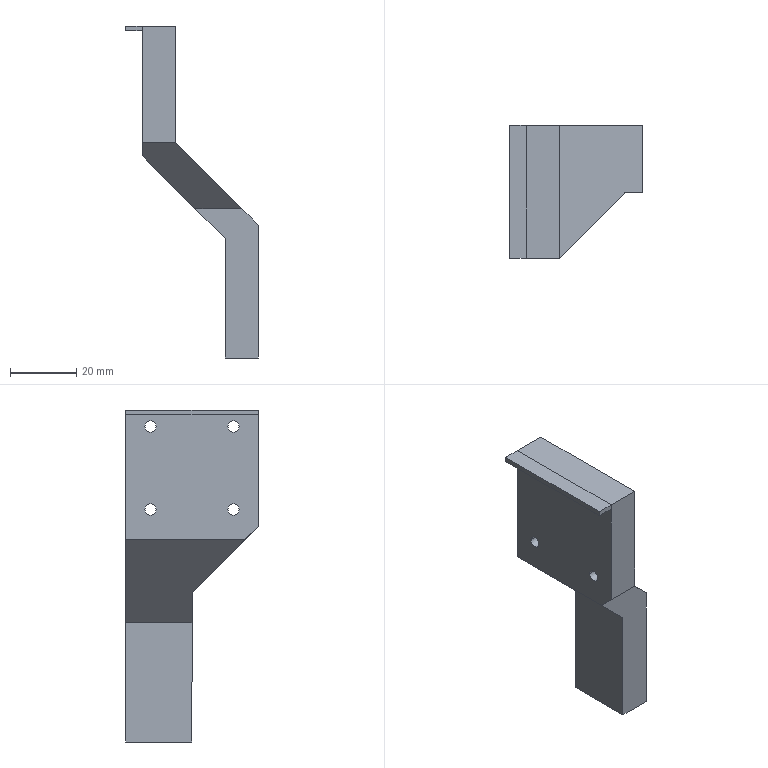Component | SolidWorks | Slider-1 | 2 solids | 26 faces | box 40 x 40 x 100 mm | volume 31677 mm3 | plane 18 | cylinder 8 | commonest cylinder face diameters 3.4 x8
STEP:
#1=COLOUR_RGB('',0.7922,0.8196,0.9333);
#2=FILL_AREA_STYLE_COLOUR('',#1);
#3=FILL_AREA_STYLE('',(#2));
#4=SURFACE_STYLE_FILL_AREA(#3);
#5=SURFACE_SIDE_STYLE('',(#4));
#6=SURFACE_STYLE_USAGE(.BOTH.,#5);
#7=PRESENTATION_STYLE_ASSIGNMENT((#6));
#8=CARTESIAN_POINT('',(-23.049,0.5207,17.664));
#9=VERTEX_POINT('',#8);
#10=CARTESIAN_POINT('',(-23.049,0.6546,17.664));
#11=VERTEX_POINT('',#10);
#12=CARTESIAN_POINT('',(-23.049,0.5877,17.664));
#13=DIRECTION('',(-1.,-0.,-0.));
#14=DIRECTION('',(0.,1.,0.));
#15=AXIS2_PLACEMENT_3D('',#12,#13,#14);
#16=CIRCLE('',#15,0.06693);
#17=EDGE_CURVE('',#9,#11,#16,.T.);
#18=ORIENTED_EDGE('',*,*,#17,.T.);
#19=CARTESIAN_POINT('',(-22.655,0.6546,17.664));
#20=VERTEX_POINT('',#19);
#21=CARTESIAN_POINT('',(-21.671,0.6546,17.664));
#22=DIRECTION('',(1.,0.,0.));
#23=VECTOR('',#22,39.37);
#24=LINE('',#21,#23);
#25=EDGE_CURVE('',#11,#20,#24,.T.);
#26=ORIENTED_EDGE('',*,*,#25,.T.);
#27=CARTESIAN_POINT('',(-22.655,0.5207,17.664));
#28=VERTEX_POINT('',#27);
#29=CARTESIAN_POINT('',(-22.655,0.5877,17.664));
#30=DIRECTION('',(-1.,-0.,-0.));
#31=DIRECTION('',(0.,-1.,0.));
#32=AXIS2_PLACEMENT_3D('',#29,#30,#31);
#33=CIRCLE('',#32,0.06693);
#34=EDGE_CURVE('',#28,#20,#33,.T.);
#35=ORIENTED_EDGE('',*,*,#34,.F.);
#36=CARTESIAN_POINT('',(-21.671,0.5207,17.664));
#37=DIRECTION('',(1.,0.,0.));
#38=VECTOR('',#37,39.37);
#39=LINE('',#36,#38);
#40=EDGE_CURVE('',#9,#28,#39,.T.);
#41=ORIENTED_EDGE('',*,*,#40,.F.);
#42=EDGE_LOOP('',(#18,#26,#35,#41));
#43=FACE_OUTER_BOUND('',#42,.T.);
#44=CARTESIAN_POINT('',(-21.671,0.5877,17.664));
#45=DIRECTION('',(1.,0.,0.));
#46=DIRECTION('',(0.,-1.,0.));
#47=AXIS2_PLACEMENT_3D('',#44,#45,#46);
#48=CYLINDRICAL_SURFACE('',#47,0.06693);
#49=ADVANCED_FACE('',(#43),#48,.F.);
#50=CARTESIAN_POINT('',(-23.049,-0.4635,17.664));
#51=VERTEX_POINT('',#50);
#52=CARTESIAN_POINT('',(-23.049,-0.3297,17.664));
#53=VERTEX_POINT('',#52);
#54=CARTESIAN_POINT('',(-23.049,-0.3966,17.664));
#55=DIRECTION('',(-1.,-0.,-0.));
#56=DIRECTION('',(0.,1.,0.));
#57=AXIS2_PLACEMENT_3D('',#54,#55,#56);
#58=CIRCLE('',#57,0.06693);
#59=EDGE_CURVE('',#51,#53,#58,.T.);
#60=ORIENTED_EDGE('',*,*,#59,.T.);
#61=CARTESIAN_POINT('',(-22.655,-0.3297,17.664));
#62=VERTEX_POINT('',#61);
#63=CARTESIAN_POINT('',(-21.671,-0.3297,17.664));
#64=DIRECTION('',(1.,0.,0.));
#65=VECTOR('',#64,39.37);
#66=LINE('',#63,#65);
#67=EDGE_CURVE('',#53,#62,#66,.T.);
#68=ORIENTED_EDGE('',*,*,#67,.T.);
#69=CARTESIAN_POINT('',(-22.655,-0.4635,17.664));
#70=VERTEX_POINT('',#69);
#71=CARTESIAN_POINT('',(-22.655,-0.3966,17.664));
#72=DIRECTION('',(-1.,-0.,-0.));
#73=DIRECTION('',(0.,-1.,0.));
#74=AXIS2_PLACEMENT_3D('',#71,#72,#73);
#75=CIRCLE('',#74,0.06693);
#76=EDGE_CURVE('',#70,#62,#75,.T.);
#77=ORIENTED_EDGE('',*,*,#76,.F.);
#78=CARTESIAN_POINT('',(-21.671,-0.4635,17.664));
#79=DIRECTION('',(1.,0.,0.));
#80=VECTOR('',#79,39.37);
#81=LINE('',#78,#80);
#82=EDGE_CURVE('',#51,#70,#81,.T.);
#83=ORIENTED_EDGE('',*,*,#82,.F.);
#84=EDGE_LOOP('',(#60,#68,#77,#83));
#85=FACE_OUTER_BOUND('',#84,.T.);
#86=CARTESIAN_POINT('',(-21.671,-0.3966,17.664));
#87=DIRECTION('',(1.,0.,0.));
#88=DIRECTION('',(0.,-1.,0.));
#89=AXIS2_PLACEMENT_3D('',#86,#87,#88);
#90=CYLINDRICAL_SURFACE('',#89,0.06693);
#91=ADVANCED_FACE('',(#85),#90,.F.);
#92=CARTESIAN_POINT('',(-23.049,0.5207,16.68));
#93=VERTEX_POINT('',#92);
#94=CARTESIAN_POINT('',(-23.049,0.6546,16.68));
#95=VERTEX_POINT('',#94);
#96=CARTESIAN_POINT('',(-23.049,0.5877,16.68));
#97=DIRECTION('',(-1.,-0.,-0.));
#98=DIRECTION('',(0.,1.,0.));
#99=AXIS2_PLACEMENT_3D('',#96,#97,#98);
#100=CIRCLE('',#99,0.06693);
#101=EDGE_CURVE('',#93,#95,#100,.T.);
#102=ORIENTED_EDGE('',*,*,#101,.T.);
#103=CARTESIAN_POINT('',(-22.655,0.6546,16.68));
#104=VERTEX_POINT('',#103);
#105=CARTESIAN_POINT('',(-21.671,0.6546,16.68));
#106=DIRECTION('',(1.,0.,0.));
#107=VECTOR('',#106,39.37);
#108=LINE('',#105,#107);
#109=EDGE_CURVE('',#95,#104,#108,.T.);
#110=ORIENTED_EDGE('',*,*,#109,.T.);
#111=CARTESIAN_POINT('',(-22.655,0.5207,16.68));
#112=VERTEX_POINT('',#111);
#113=CARTESIAN_POINT('',(-22.655,0.5877,16.68));
#114=DIRECTION('',(-1.,-0.,-0.));
#115=DIRECTION('',(0.,-1.,0.));
#116=AXIS2_PLACEMENT_3D('',#113,#114,#115);
#117=CIRCLE('',#116,0.06693);
#118=EDGE_CURVE('',#112,#104,#117,.T.);
#119=ORIENTED_EDGE('',*,*,#118,.F.);
#120=CARTESIAN_POINT('',(-21.671,0.5207,16.68));
#121=DIRECTION('',(1.,0.,0.));
#122=VECTOR('',#121,39.37);
#123=LINE('',#120,#122);
#124=EDGE_CURVE('',#93,#112,#123,.T.);
#125=ORIENTED_EDGE('',*,*,#124,.F.);
#126=EDGE_LOOP('',(#102,#110,#119,#125));
#127=FACE_OUTER_BOUND('',#126,.T.);
#128=CARTESIAN_POINT('',(-21.671,0.5877,16.68));
#129=DIRECTION('',(1.,0.,0.));
#130=DIRECTION('',(0.,-1.,0.));
#131=AXIS2_PLACEMENT_3D('',#128,#129,#130);
#132=CYLINDRICAL_SURFACE('',#131,0.06693);
#133=ADVANCED_FACE('',(#127),#132,.F.);
#134=CARTESIAN_POINT('',(-23.049,-0.4635,16.68));
#135=VERTEX_POINT('',#134);
#136=CARTESIAN_POINT('',(-23.049,-0.3297,16.68));
#137=VERTEX_POINT('',#136);
#138=CARTESIAN_POINT('',(-23.049,-0.3966,16.68));
#139=DIRECTION('',(-1.,-0.,-0.));
#140=DIRECTION('',(0.,1.,0.));
#141=AXIS2_PLACEMENT_3D('',#138,#139,#140);
#142=CIRCLE('',#141,0.06693);
#143=EDGE_CURVE('',#135,#137,#142,.T.);
#144=ORIENTED_EDGE('',*,*,#143,.T.);
#145=CARTESIAN_POINT('',(-22.655,-0.3297,16.68));
#146=VERTEX_POINT('',#145);
#147=CARTESIAN_POINT('',(-21.671,-0.3297,16.68));
#148=DIRECTION('',(1.,0.,0.));
#149=VECTOR('',#148,39.37);
#150=LINE('',#147,#149);
#151=EDGE_CURVE('',#137,#146,#150,.T.);
#152=ORIENTED_EDGE('',*,*,#151,.T.);
#153=CARTESIAN_POINT('',(-22.655,-0.4635,16.68));
#154=VERTEX_POINT('',#153);
#155=CARTESIAN_POINT('',(-22.655,-0.3966,16.68));
#156=DIRECTION('',(-1.,-0.,-0.));
#157=DIRECTION('',(0.,-1.,0.));
#158=AXIS2_PLACEMENT_3D('',#155,#156,#157);
#159=CIRCLE('',#158,0.06693);
#160=EDGE_CURVE('',#154,#146,#159,.T.);
#161=ORIENTED_EDGE('',*,*,#160,.F.);
#162=CARTESIAN_POINT('',(-21.671,-0.4635,16.68));
#163=DIRECTION('',(1.,0.,0.));
#164=VECTOR('',#163,39.37);
#165=LINE('',#162,#164);
#166=EDGE_CURVE('',#135,#154,#165,.T.);
#167=ORIENTED_EDGE('',*,*,#166,.F.);
#168=EDGE_LOOP('',(#144,#152,#161,#167));
#169=FACE_OUTER_BOUND('',#168,.T.);
#170=CARTESIAN_POINT('',(-21.671,-0.3966,16.68));
#171=DIRECTION('',(1.,0.,0.));
#172=DIRECTION('',(0.,-1.,0.));
#173=AXIS2_PLACEMENT_3D('',#170,#171,#172);
#174=CYLINDRICAL_SURFACE('',#173,0.06693);
#175=ADVANCED_FACE('',(#169),#174,.F.);
#176=CARTESIAN_POINT('',(-22.655,0.8829,17.861));
#177=VERTEX_POINT('',#176);
#178=CARTESIAN_POINT('',(-22.655,0.8829,16.483));
#179=VERTEX_POINT('',#178);
#180=CARTESIAN_POINT('',(-22.655,0.8829,17.861));
#181=DIRECTION('',(0.,0.,-1.));
#182=VECTOR('',#181,39.37);
#183=LINE('',#180,#182);
#184=EDGE_CURVE('',#177,#179,#183,.T.);
#185=ORIENTED_EDGE('',*,*,#184,.T.);
#186=CARTESIAN_POINT('',(-21.671,0.8829,15.499));
#187=VERTEX_POINT('',#186);
#188=CARTESIAN_POINT('',(-22.655,0.8829,16.483));
#189=DIRECTION('',(0.7071,0.,-0.7071));
#190=VECTOR('',#189,39.37);
#191=LINE('',#188,#190);
#192=EDGE_CURVE('',#179,#187,#191,.T.);
#193=ORIENTED_EDGE('',*,*,#192,.T.);
#194=CARTESIAN_POINT('',(-21.671,0.8829,13.924));
#195=VERTEX_POINT('',#194);
#196=CARTESIAN_POINT('',(-21.671,0.8829,17.861));
#197=DIRECTION('',(-0.,-0.,1.));
#198=VECTOR('',#197,39.37);
#199=LINE('',#196,#198);
#200=EDGE_CURVE('',#195,#187,#199,.T.);
#201=ORIENTED_EDGE('',*,*,#200,.F.);
#202=CARTESIAN_POINT('',(-22.065,0.8829,13.924));
#203=VERTEX_POINT('',#202);
#204=CARTESIAN_POINT('',(-21.671,0.8829,13.924));
#205=DIRECTION('',(-1.,-0.,-0.));
#206=VECTOR('',#205,39.37);
#207=LINE('',#204,#206);
#208=EDGE_CURVE('',#195,#203,#207,.T.);
#209=ORIENTED_EDGE('',*,*,#208,.T.);
#210=CARTESIAN_POINT('',(-22.065,0.8829,15.336));
#211=VERTEX_POINT('',#210);
#212=CARTESIAN_POINT('',(-22.065,0.8829,13.924));
#213=DIRECTION('',(-0.,-0.,1.));
#214=VECTOR('',#213,39.37);
#215=LINE('',#212,#214);
#216=EDGE_CURVE('',#203,#211,#215,.T.);
#217=ORIENTED_EDGE('',*,*,#216,.T.);
#218=CARTESIAN_POINT('',(-23.049,0.8829,16.32));
#219=VERTEX_POINT('',#218);
#220=CARTESIAN_POINT('',(-22.065,0.8829,15.336));
#221=DIRECTION('',(-0.7071,-0.,0.7071));
#222=VECTOR('',#221,39.37);
#223=LINE('',#220,#222);
#224=EDGE_CURVE('',#211,#219,#223,.T.);
#225=ORIENTED_EDGE('',*,*,#224,.T.);
#226=CARTESIAN_POINT('',(-23.049,0.8829,17.861));
#227=VERTEX_POINT('',#226);
#228=CARTESIAN_POINT('',(-23.049,0.8829,17.861));
#229=DIRECTION('',(-0.,-0.,1.));
#230=VECTOR('',#229,39.37);
#231=LINE('',#228,#230);
#232=EDGE_CURVE('',#219,#227,#231,.T.);
#233=ORIENTED_EDGE('',*,*,#232,.T.);
#234=CARTESIAN_POINT('',(-21.671,0.8829,17.861));
#235=DIRECTION('',(-1.,-0.,-0.));
#236=VECTOR('',#235,39.37);
#237=LINE('',#234,#236);
#238=EDGE_CURVE('',#177,#227,#237,.T.);
#239=ORIENTED_EDGE('',*,*,#238,.F.);
#240=EDGE_LOOP('',(#185,#193,#201,#209,#217,#225,#233,#239));
#241=FACE_OUTER_BOUND('',#240,.T.);
#242=CARTESIAN_POINT('',(-21.671,0.8829,17.861));
#243=DIRECTION('',(0.,-1.,-0.));
#244=DIRECTION('',(-1.,-0.,-0.));
#245=AXIS2_PLACEMENT_3D('',#242,#243,#244);
#246=PLANE('',#245);
#247=ADVANCED_FACE('',(#241),#246,.F.);
#248=CARTESIAN_POINT('',(-22.655,-0.6919,17.861));
#249=VERTEX_POINT('',#248);
#250=CARTESIAN_POINT('',(-22.655,-1.282,17.861));
#251=DIRECTION('',(-0.,1.,0.));
#252=VECTOR('',#251,39.37);
#253=LINE('',#250,#252);
#254=EDGE_CURVE('',#249,#177,#253,.T.);
#255=ORIENTED_EDGE('',*,*,#254,.T.);
#256=ORIENTED_EDGE('',*,*,#238,.T.);
#257=CARTESIAN_POINT('',(-23.049,-0.6919,17.861));
#258=VERTEX_POINT('',#257);
#259=CARTESIAN_POINT('',(-23.049,0.8829,17.861));
#260=DIRECTION('',(0.,-1.,-0.));
#261=VECTOR('',#260,39.37);
#262=LINE('',#259,#261);
#263=EDGE_CURVE('',#227,#258,#262,.T.);
#264=ORIENTED_EDGE('',*,*,#263,.T.);
#265=CARTESIAN_POINT('',(-21.671,-0.6919,17.861));
#266=DIRECTION('',(-1.,-0.,-0.));
#267=VECTOR('',#266,39.37);
#268=LINE('',#265,#267);
#269=EDGE_CURVE('',#249,#258,#268,.T.);
#270=ORIENTED_EDGE('',*,*,#269,.F.);
#271=EDGE_LOOP('',(#255,#256,#264,#270));
#272=FACE_OUTER_BOUND('',#271,.T.);
#273=CARTESIAN_POINT('',(-21.671,0.8829,17.861));
#274=DIRECTION('',(0.,0.,-1.));
#275=DIRECTION('',(1.,0.,0.));
#276=AXIS2_PLACEMENT_3D('',#273,#274,#275);
#277=PLANE('',#276);
#278=ADVANCED_FACE('',(#272),#277,.F.);
#279=CARTESIAN_POINT('',(-22.655,-0.6919,16.483));
#280=VERTEX_POINT('',#279);
#281=CARTESIAN_POINT('',(-22.655,-0.6919,17.861));
#282=DIRECTION('',(0.,0.,-1.));
#283=VECTOR('',#282,39.37);
#284=LINE('',#281,#283);
#285=EDGE_CURVE('',#249,#280,#284,.T.);
#286=ORIENTED_EDGE('',*,*,#285,.F.);
#287=ORIENTED_EDGE('',*,*,#269,.T.);
#288=CARTESIAN_POINT('',(-23.049,-0.6919,16.483));
#289=VERTEX_POINT('',#288);
#290=CARTESIAN_POINT('',(-23.049,-0.6919,17.861));
#291=DIRECTION('',(0.,0.,-1.));
#292=VECTOR('',#291,39.37);
#293=LINE('',#290,#292);
#294=EDGE_CURVE('',#258,#289,#293,.T.);
#295=ORIENTED_EDGE('',*,*,#294,.T.);
#296=CARTESIAN_POINT('',(-21.671,-0.6919,16.483));
#297=DIRECTION('',(-1.,-0.,-0.));
#298=VECTOR('',#297,39.37);
#299=LINE('',#296,#298);
#300=EDGE_CURVE('',#280,#289,#299,.T.);
#301=ORIENTED_EDGE('',*,*,#300,.F.);
#302=EDGE_LOOP('',(#286,#287,#295,#301));
#303=FACE_OUTER_BOUND('',#302,.T.);
#304=CARTESIAN_POINT('',(-21.671,-0.6919,17.861));
#305=DIRECTION('',(-0.,1.,0.));
#306=DIRECTION('',(-0.,-0.,1.));
#307=AXIS2_PLACEMENT_3D('',#304,#305,#306);
#308=PLANE('',#307);
#309=ADVANCED_FACE('',(#303),#308,.F.);
#310=CARTESIAN_POINT('',(-21.868,0.09553,15.696));
#311=VERTEX_POINT('',#310);
#312=CARTESIAN_POINT('',(-21.671,0.09553,15.499));
#313=VERTEX_POINT('',#312);
#314=CARTESIAN_POINT('',(-22.163,0.09553,15.991));
#315=DIRECTION('',(0.7071,0.,-0.7071));
#316=VECTOR('',#315,39.37);
#317=LINE('',#314,#316);
#318=EDGE_CURVE('',#311,#313,#317,.T.);
#319=ORIENTED_EDGE('',*,*,#318,.F.);
#320=CARTESIAN_POINT('',(-22.425,0.09553,15.696));
#321=VERTEX_POINT('',#320);
#322=CARTESIAN_POINT('',(-23.049,0.09553,15.696));
#323=DIRECTION('',(-1.,-0.,-0.));
#324=VECTOR('',#323,39.37);
#325=LINE('',#322,#324);
#326=EDGE_CURVE('',#311,#321,#325,.T.);
#327=ORIENTED_EDGE('',*,*,#326,.T.);
#328=CARTESIAN_POINT('',(-22.065,0.09553,15.336));
#329=VERTEX_POINT('',#328);
#330=CARTESIAN_POINT('',(-22.442,0.09553,15.712));
#331=DIRECTION('',(-0.7071,-0.,0.7071));
#332=VECTOR('',#331,39.37);
#333=LINE('',#330,#332);
#334=EDGE_CURVE('',#329,#321,#333,.T.);
#335=ORIENTED_EDGE('',*,*,#334,.F.);
#336=CARTESIAN_POINT('',(-22.065,0.09553,13.924));
#337=VERTEX_POINT('',#336);
#338=CARTESIAN_POINT('',(-22.065,0.09553,16.483));
#339=DIRECTION('',(-0.,-0.,1.));
#340=VECTOR('',#339,39.37);
#341=LINE('',#338,#340);
#342=EDGE_CURVE('',#337,#329,#341,.T.);
#343=ORIENTED_EDGE('',*,*,#342,.F.);
#344=CARTESIAN_POINT('',(-21.671,0.09553,13.924));
#345=VERTEX_POINT('',#344);
#346=CARTESIAN_POINT('',(-21.671,0.09553,13.924));
#347=DIRECTION('',(-1.,-0.,-0.));
#348=VECTOR('',#347,39.37);
#349=LINE('',#346,#348);
#350=EDGE_CURVE('',#345,#337,#349,.T.);
#351=ORIENTED_EDGE('',*,*,#350,.F.);
#352=CARTESIAN_POINT('',(-21.671,0.09553,16.483));
#353=DIRECTION('',(0.,0.,-1.));
#354=VECTOR('',#353,39.37);
#355=LINE('',#352,#354);
#356=EDGE_CURVE('',#313,#345,#355,.T.);
#357=ORIENTED_EDGE('',*,*,#356,.F.);
#358=EDGE_LOOP('',(#319,#327,#335,#343,#351,#357));
#359=FACE_OUTER_BOUND('',#358,.T.);
#360=CARTESIAN_POINT('',(-21.671,0.09553,16.483));
#361=DIRECTION('',(-0.,1.,0.));
#362=DIRECTION('',(1.,0.,0.));
#363=AXIS2_PLACEMENT_3D('',#360,#361,#362);
#364=PLANE('',#363);
#365=ADVANCED_FACE('',(#359),#364,.F.);
#366=CARTESIAN_POINT('',(-22.065,-1.282,13.924));
#367=DIRECTION('',(-0.,1.,0.));
#368=VECTOR('',#367,39.37);
#369=LINE('',#366,#368);
#370=EDGE_CURVE('',#337,#203,#369,.T.);
#371=ORIENTED_EDGE('',*,*,#370,.T.);
#372=ORIENTED_EDGE('',*,*,#208,.F.);
#373=CARTESIAN_POINT('',(-21.671,0.8829,13.924));
#374=DIRECTION('',(-0.,1.,0.));
#375=VECTOR('',#374,39.37);
#376=LINE('',#373,#375);
#377=EDGE_CURVE('',#345,#195,#376,.T.);
#378=ORIENTED_EDGE('',*,*,#377,.F.);
#379=ORIENTED_EDGE('',*,*,#350,.T.);
#380=EDGE_LOOP('',(#371,#372,#378,#379));
#381=FACE_OUTER_BOUND('',#380,.T.);
#382=CARTESIAN_POINT('',(-21.671,0.8829,13.924));
#383=DIRECTION('',(-0.,-0.,1.));
#384=DIRECTION('',(-1.,-0.,-0.));
#385=AXIS2_PLACEMENT_3D('',#382,#383,#384);
#386=PLANE('',#385);
#387=ADVANCED_FACE('',(#381),#386,.F.);
#388=CARTESIAN_POINT('',(-21.671,-1.282,15.499));
#389=DIRECTION('',(-0.,1.,0.));
#390=VECTOR('',#389,39.37);
#391=LINE('',#388,#390);
#392=EDGE_CURVE('',#313,#187,#391,.T.);
#393=ORIENTED_EDGE('',*,*,#392,.F.);
#394=ORIENTED_EDGE('',*,*,#356,.T.);
#395=ORIENTED_EDGE('',*,*,#377,.T.);
#396=ORIENTED_EDGE('',*,*,#200,.T.);
#397=EDGE_LOOP('',(#393,#394,#395,#396));
#398=FACE_OUTER_BOUND('',#397,.T.);
#399=CARTESIAN_POINT('',(-21.671,0.1353,17.169));
#400=DIRECTION('',(-1.,-0.,-0.));
#401=DIRECTION('',(-0.,1.,0.));
#402=AXIS2_PLACEMENT_3D('',#399,#400,#401);
#403=PLANE('',#402);
#404=ADVANCED_FACE('',(#398),#403,.F.);
#405=ORIENTED_EDGE('',*,*,#17,.F.);
#406=CARTESIAN_POINT('',(-23.049,0.5877,17.664));
#407=DIRECTION('',(-1.,-0.,-0.));
#408=DIRECTION('',(0.,1.,0.));
#409=AXIS2_PLACEMENT_3D('',#406,#407,#408);
#410=CIRCLE('',#409,0.06693);
#411=EDGE_CURVE('',#11,#9,#410,.T.);
#412=ORIENTED_EDGE('',*,*,#411,.F.);
#413=EDGE_LOOP('',(#405,#412));
#414=FACE_BOUND('',#413,.T.);
#415=ORIENTED_EDGE('',*,*,#59,.F.);
#416=CARTESIAN_POINT('',(-23.049,-0.3966,17.664));
#417=DIRECTION('',(-1.,-0.,-0.));
#418=DIRECTION('',(0.,1.,0.));
#419=AXIS2_PLACEMENT_3D('',#416,#417,#418);
#420=CIRCLE('',#419,0.06693);
#421=EDGE_CURVE('',#53,#51,#420,.T.);
#422=ORIENTED_EDGE('',*,*,#421,.F.);
#423=EDGE_LOOP('',(#415,#422));
#424=FACE_BOUND('',#423,.T.);
#425=ORIENTED_EDGE('',*,*,#101,.F.);
#426=CARTESIAN_POINT('',(-23.049,0.5877,16.68));
#427=DIRECTION('',(-1.,-0.,-0.));
#428=DIRECTION('',(0.,1.,0.));
#429=AXIS2_PLACEMENT_3D('',#426,#427,#428);
#430=CIRCLE('',#429,0.06693);
#431=EDGE_CURVE('',#95,#93,#430,.T.);
#432=ORIENTED_EDGE('',*,*,#431,.F.);
#433=EDGE_LOOP('',(#425,#432));
#434=FACE_BOUND('',#433,.T.);
#435=ORIENTED_EDGE('',*,*,#143,.F.);
#436=CARTESIAN_POINT('',(-23.049,-0.3966,16.68));
#437=DIRECTION('',(-1.,-0.,-0.));
#438=DIRECTION('',(0.,1.,0.));
#439=AXIS2_PLACEMENT_3D('',#436,#437,#438);
#440=CIRCLE('',#439,0.06693);
#441=EDGE_CURVE('',#137,#135,#440,.T.);
#442=ORIENTED_EDGE('',*,*,#441,.F.);
#443=EDGE_LOOP('',(#435,#442));
#444=FACE_BOUND('',#443,.T.);
#445=ORIENTED_EDGE('',*,*,#232,.F.);
#446=CARTESIAN_POINT('',(-23.049,-0.5288,16.32));
#447=VERTEX_POINT('',#446);
#448=CARTESIAN_POINT('',(-23.049,-1.282,16.32));
#449=DIRECTION('',(-0.,1.,0.));
#450=VECTOR('',#449,39.37);
#451=LINE('',#448,#450);
#452=EDGE_CURVE('',#447,#219,#451,.T.);
#453=ORIENTED_EDGE('',*,*,#452,.F.);
#454=CARTESIAN_POINT('',(-23.049,0.09553,15.696));
#455=DIRECTION('',(-0.,-0.7071,0.7071));
#456=VECTOR('',#455,39.37);
#457=LINE('',#454,#456);
#458=EDGE_CURVE('',#447,#289,#457,.T.);
#459=ORIENTED_EDGE('',*,*,#458,.T.);
#460=ORIENTED_EDGE('',*,*,#294,.F.);
#461=ORIENTED_EDGE('',*,*,#263,.F.);
#462=EDGE_LOOP('',(#445,#453,#459,#460,#461));
#463=FACE_OUTER_BOUND('',#462,.T.);
#464=CARTESIAN_POINT('',(-23.049,0.1353,17.169));
#465=DIRECTION('',(-1.,-0.,-0.));
#466=DIRECTION('',(-0.,1.,0.));
#467=AXIS2_PLACEMENT_3D('',#464,#465,#466);
#468=PLANE('',#467);
#469=ADVANCED_FACE('',(#414,#424,#434,#444,#463),#468,.T.);
#470=CARTESIAN_POINT('',(-21.802,0.1611,15.63));
#471=DIRECTION('',(0.5774,0.5774,-0.5774));
#472=VECTOR('',#471,39.37);
#473=LINE('',#470,#472);
#474=EDGE_CURVE('',#280,#311,#473,.T.);
#475=ORIENTED_EDGE('',*,*,#474,.F.);
#476=ORIENTED_EDGE('',*,*,#300,.T.);
#477=ORIENTED_EDGE('',*,*,#458,.F.);
#478=CARTESIAN_POINT('',(-22.174,0.3467,15.444));
#479=DIRECTION('',(-0.5774,-0.5774,0.5774));
#480=VECTOR('',#479,39.37);
#481=LINE('',#478,#480);
#482=EDGE_CURVE('',#321,#447,#481,.T.);
#483=ORIENTED_EDGE('',*,*,#482,.F.);
#484=ORIENTED_EDGE('',*,*,#326,.F.);
#485=EDGE_LOOP('',(#475,#476,#477,#483,#484));
#486=FACE_OUTER_BOUND('',#485,.T.);
#487=CARTESIAN_POINT('',(-21.671,0.09553,15.696));
#488=DIRECTION('',(0.,-0.7071,-0.7071));
#489=DIRECTION('',(1.,0.,0.));
#490=AXIS2_PLACEMENT_3D('',#487,#488,#489);
#491=PLANE('',#490);
#492=ADVANCED_FACE('',(#486),#491,.T.);
#493=ORIENTED_EDGE('',*,*,#151,.F.);
#494=ORIENTED_EDGE('',*,*,#441,.T.);
#495=ORIENTED_EDGE('',*,*,#166,.T.);
#496=CARTESIAN_POINT('',(-22.655,-0.3966,16.68));
#497=DIRECTION('',(-1.,-0.,-0.));
#498=DIRECTION('',(0.,-1.,0.));
#499=AXIS2_PLACEMENT_3D('',#496,#497,#498);
#500=CIRCLE('',#499,0.06693);
#501=EDGE_CURVE('',#146,#154,#500,.T.);
#502=ORIENTED_EDGE('',*,*,#501,.F.);
#503=EDGE_LOOP('',(#493,#494,#495,#502));
#504=FACE_OUTER_BOUND('',#503,.T.);
#505=CARTESIAN_POINT('',(-21.671,-0.3966,16.68));
#506=DIRECTION('',(1.,0.,0.));
#507=DIRECTION('',(0.,-1.,0.));
#508=AXIS2_PLACEMENT_3D('',#505,#506,#507);
#509=CYLINDRICAL_SURFACE('',#508,0.06693);
#510=ADVANCED_FACE('',(#504),#509,.F.);
#511=ORIENTED_EDGE('',*,*,#109,.F.);
#512=ORIENTED_EDGE('',*,*,#431,.T.);
#513=ORIENTED_EDGE('',*,*,#124,.T.);
#514=CARTESIAN_POINT('',(-22.655,0.5877,16.68));
#515=DIRECTION('',(-1.,-0.,-0.));
#516=DIRECTION('',(0.,-1.,0.));
#517=AXIS2_PLACEMENT_3D('',#514,#515,#516);
#518=CIRCLE('',#517,0.06693);
#519=EDGE_CURVE('',#104,#112,#518,.T.);
#520=ORIENTED_EDGE('',*,*,#519,.F.);
#521=EDGE_LOOP('',(#511,#512,#513,#520));
#522=FACE_OUTER_BOUND('',#521,.T.);
#523=CARTESIAN_POINT('',(-21.671,0.5877,16.68));
#524=DIRECTION('',(1.,0.,0.));
#525=DIRECTION('',(0.,-1.,0.));
#526=AXIS2_PLACEMENT_3D('',#523,#524,#525);
#527=CYLINDRICAL_SURFACE('',#526,0.06693);
#528=ADVANCED_FACE('',(#522),#527,.F.);
#529=ORIENTED_EDGE('',*,*,#67,.F.);
#530=ORIENTED_EDGE('',*,*,#421,.T.);
#531=ORIENTED_EDGE('',*,*,#82,.T.);
#532=CARTESIAN_POINT('',(-22.655,-0.3966,17.664));
#533=DIRECTION('',(-1.,-0.,-0.));
#534=DIRECTION('',(0.,-1.,0.));
#535=AXIS2_PLACEMENT_3D('',#532,#533,#534);
#536=CIRCLE('',#535,0.06693);
#537=EDGE_CURVE('',#62,#70,#536,.T.);
#538=ORIENTED_EDGE('',*,*,#537,.F.);
#539=EDGE_LOOP('',(#529,#530,#531,#538));
#540=FACE_OUTER_BOUND('',#539,.T.);
#541=CARTESIAN_POINT('',(-21.671,-0.3966,17.664));
#542=DIRECTION('',(1.,0.,0.));
#543=DIRECTION('',(0.,-1.,0.));
#544=AXIS2_PLACEMENT_3D('',#541,#542,#543);
#545=CYLINDRICAL_SURFACE('',#544,0.06693);
#546=ADVANCED_FACE('',(#540),#545,.F.);
#547=ORIENTED_EDGE('',*,*,#25,.F.);
#548=ORIENTED_EDGE('',*,*,#411,.T.);
#549=ORIENTED_EDGE('',*,*,#40,.T.);
#550=CARTESIAN_POINT('',(-22.655,0.5877,17.664));
#551=DIRECTION('',(-1.,-0.,-0.));
#552=DIRECTION('',(0.,-1.,0.));
#553=AXIS2_PLACEMENT_3D('',#550,#551,#552);
#554=CIRCLE('',#553,0.06693);
#555=EDGE_CURVE('',#20,#28,#554,.T.);
#556=ORIENTED_EDGE('',*,*,#555,.F.);
#557=EDGE_LOOP('',(#547,#548,#549,#556));
#558=FACE_OUTER_BOUND('',#557,.T.);
#559=CARTESIAN_POINT('',(-21.671,0.5877,17.664));
#560=DIRECTION('',(1.,0.,0.));
#561=DIRECTION('',(0.,-1.,0.));
#562=AXIS2_PLACEMENT_3D('',#559,#560,#561);
#563=CYLINDRICAL_SURFACE('',#562,0.06693);
#564=ADVANCED_FACE('',(#558),#563,.F.);
#565=ORIENTED_EDGE('',*,*,#318,.T.);
#566=ORIENTED_EDGE('',*,*,#392,.T.);
#567=ORIENTED_EDGE('',*,*,#192,.F.);
#568=CARTESIAN_POINT('',(-22.655,-1.282,16.483));
#569=DIRECTION('',(-0.,1.,0.));
#570=VECTOR('',#569,39.37);
#571=LINE('',#568,#570);
#572=EDGE_CURVE('',#280,#179,#571,.T.);
#573=ORIENTED_EDGE('',*,*,#572,.F.);
#574=ORIENTED_EDGE('',*,*,#474,.T.);
#575=EDGE_LOOP('',(#565,#566,#567,#573,#574));
#576=FACE_OUTER_BOUND('',#575,.T.);
#577=CARTESIAN_POINT('',(-22.655,-1.282,16.483));
#578=DIRECTION('',(0.7071,-0.,0.7071));
#579=DIRECTION('',(-0.7071,-0.,0.7071));
#580=AXIS2_PLACEMENT_3D('',#577,#578,#579);
#581=PLANE('',#580);
#582=ADVANCED_FACE('',(#576),#581,.T.);
#583=ORIENTED_EDGE('',*,*,#160,.T.);
#584=ORIENTED_EDGE('',*,*,#501,.T.);
#585=EDGE_LOOP('',(#583,#584));
#586=FACE_BOUND('',#585,.T.);
#587=ORIENTED_EDGE('',*,*,#118,.T.);
#588=ORIENTED_EDGE('',*,*,#519,.T.);
#589=EDGE_LOOP('',(#587,#588));
#590=FACE_BOUND('',#589,.T.);
#591=ORIENTED_EDGE('',*,*,#76,.T.);
#592=ORIENTED_EDGE('',*,*,#537,.T.);
#593=EDGE_LOOP('',(#591,#592));
#594=FACE_BOUND('',#593,.T.);
#595=ORIENTED_EDGE('',*,*,#34,.T.);
#596=ORIENTED_EDGE('',*,*,#555,.T.);
#597=EDGE_LOOP('',(#595,#596));
#598=FACE_BOUND('',#597,.T.);
#599=ORIENTED_EDGE('',*,*,#285,.T.);
#600=ORIENTED_EDGE('',*,*,#572,.T.);
#601=ORIENTED_EDGE('',*,*,#184,.F.);
#602=ORIENTED_EDGE('',*,*,#254,.F.);
#603=EDGE_LOOP('',(#599,#600,#601,#602));
#604=FACE_OUTER_BOUND('',#603,.T.);
#605=CARTESIAN_POINT('',(-22.655,-1.282,17.861));
#606=DIRECTION('',(1.,0.,0.));
#607=DIRECTION('',(0.,-1.,-0.));
#608=AXIS2_PLACEMENT_3D('',#605,#606,#607);
#609=PLANE('',#608);
#610=ADVANCED_FACE('',(#586,#590,#594,#598,#604),#609,.T.);
#611=ORIENTED_EDGE('',*,*,#342,.T.);
#612=CARTESIAN_POINT('',(-22.065,-1.282,15.336));
#613=DIRECTION('',(-0.,1.,0.));
#614=VECTOR('',#613,39.37);
#615=LINE('',#612,#614);
#616=EDGE_CURVE('',#329,#211,#615,.T.);
#617=ORIENTED_EDGE('',*,*,#616,.T.);
#618=ORIENTED_EDGE('',*,*,#216,.F.);
#619=ORIENTED_EDGE('',*,*,#370,.F.);
#620=EDGE_LOOP('',(#611,#617,#618,#619));
#621=FACE_OUTER_BOUND('',#620,.T.);
#622=CARTESIAN_POINT('',(-22.065,-1.282,13.924));
#623=DIRECTION('',(-1.,-0.,-0.));
#624=DIRECTION('',(0.,0.,-1.));
#625=AXIS2_PLACEMENT_3D('',#622,#623,#624);
#626=PLANE('',#625);
#627=ADVANCED_FACE('',(#621),#626,.T.);
#628=ORIENTED_EDGE('',*,*,#334,.T.);
#629=ORIENTED_EDGE('',*,*,#482,.T.);
#630=ORIENTED_EDGE('',*,*,#452,.T.);
#631=ORIENTED_EDGE('',*,*,#224,.F.);
#632=ORIENTED_EDGE('',*,*,#616,.F.);
#633=EDGE_LOOP('',(#628,#629,#630,#631,#632));
#634=FACE_OUTER_BOUND('',#633,.T.);
#635=CARTESIAN_POINT('',(-22.065,-1.282,15.336));
#636=DIRECTION('',(-0.7071,0.,-0.7071));
#637=DIRECTION('',(0.7071,0.,-0.7071));
#638=AXIS2_PLACEMENT_3D('',#635,#636,#637);
#639=PLANE('',#638);
#640=ADVANCED_FACE('',(#634),#639,.T.);
#641=CLOSED_SHELL('',(#49,#91,#133,#175,#247,#278,#309,#365,#387,#404,#469,#492,#510,#528,#546,#564,#582,#610,#627,#640));
#642=MANIFOLD_SOLID_BREP('',#641);
#643=STYLED_ITEM('',(#7),#642);
#644=(LENGTH_UNIT()NAMED_UNIT(*)SI_UNIT($,.METRE.));
#645=LENGTH_MEASURE_WITH_UNIT(LENGTH_MEASURE(0.0254),#644);
#646=DIMENSIONAL_EXPONENTS(1.,0.,0.,0.,0.,0.,0.);
#647=(CONVERSION_BASED_UNIT('',#645)LENGTH_UNIT()NAMED_UNIT(#646));
#648=UNCERTAINTY_MEASURE_WITH_UNIT(LENGTH_MEASURE(0.00001),#647,'','');
#649=(NAMED_UNIT(*)PLANE_ANGLE_UNIT()SI_UNIT($,.RADIAN.));
#650=(NAMED_UNIT(*)SI_UNIT($,.STERADIAN.)SOLID_ANGLE_UNIT());
#651=(GEOMETRIC_REPRESENTATION_CONTEXT(3)GLOBAL_UNCERTAINTY_ASSIGNED_CONTEXT((#648))GLOBAL_UNIT_ASSIGNED_CONTEXT((#647,#649,#650))REPRESENTATION_CONTEXT('',''));
#652=MECHANICAL_DESIGN_GEOMETRIC_PRESENTATION_REPRESENTATION('',(#643),#651);
#653=PRESENTATION_LAYER_ASSIGNMENT('','',(#643));
#654=CARTESIAN_POINT('',(-23.049,0.8829,17.861));
#655=VERTEX_POINT('',#654);
#656=CARTESIAN_POINT('',(-23.049,0.8829,17.802));
#657=VERTEX_POINT('',#656);
#658=CARTESIAN_POINT('',(-23.049,0.8829,17.861));
#659=DIRECTION('',(0.,0.,-1.));
#660=VECTOR('',#659,39.37);
#661=LINE('',#658,#660);
#662=EDGE_CURVE('',#655,#657,#661,.T.);
#663=ORIENTED_EDGE('',*,*,#662,.T.);
#664=CARTESIAN_POINT('',(-23.246,0.8829,17.802));
#665=VERTEX_POINT('',#664);
#666=CARTESIAN_POINT('',(-23.246,0.8829,17.802));
#667=DIRECTION('',(1.,0.,0.));
#668=VECTOR('',#667,39.37);
#669=LINE('',#666,#668);
#670=EDGE_CURVE('',#665,#657,#669,.T.);
#671=ORIENTED_EDGE('',*,*,#670,.F.);
#672=CARTESIAN_POINT('',(-23.246,0.8829,17.861));
#673=VERTEX_POINT('',#672);
#674=CARTESIAN_POINT('',(-23.246,0.8829,17.861));
#675=DIRECTION('',(0.,0.,-1.));
#676=VECTOR('',#675,39.37);
#677=LINE('',#674,#676);
#678=EDGE_CURVE('',#673,#665,#677,.T.);
#679=ORIENTED_EDGE('',*,*,#678,.F.);
#680=CARTESIAN_POINT('',(-23.246,0.8829,17.861));
#681=DIRECTION('',(1.,0.,0.));
#682=VECTOR('',#681,39.37);
#683=LINE('',#680,#682);
#684=EDGE_CURVE('',#673,#655,#683,.T.);
#685=ORIENTED_EDGE('',*,*,#684,.T.);
#686=EDGE_LOOP('',(#663,#671,#679,#685));
#687=FACE_OUTER_BOUND('',#686,.T.);
#688=CARTESIAN_POINT('',(-23.246,0.8829,17.861));
#689=DIRECTION('',(0.,-1.,-0.));
#690=DIRECTION('',(-1.,-0.,-0.));
#691=AXIS2_PLACEMENT_3D('',#688,#689,#690);
#692=PLANE('',#691);
#693=ADVANCED_FACE('',(#687),#692,.F.);
#694=CARTESIAN_POINT('',(-23.049,-0.6919,17.802));
#695=VERTEX_POINT('',#694);
#696=CARTESIAN_POINT('',(-23.049,0.8829,17.802));
#697=DIRECTION('',(0.,-1.,-0.));
#698=VECTOR('',#697,39.37);
#699=LINE('',#696,#698);
#700=EDGE_CURVE('',#657,#695,#699,.T.);
#701=ORIENTED_EDGE('',*,*,#700,.T.);
#702=CARTESIAN_POINT('',(-23.246,-0.6919,17.802));
#703=VERTEX_POINT('',#702);
#704=CARTESIAN_POINT('',(-23.246,-0.6919,17.802));
#705=DIRECTION('',(1.,0.,0.));
#706=VECTOR('',#705,39.37);
#707=LINE('',#704,#706);
#708=EDGE_CURVE('',#703,#695,#707,.T.);
#709=ORIENTED_EDGE('',*,*,#708,.F.);
#710=CARTESIAN_POINT('',(-23.246,0.8829,17.802));
#711=DIRECTION('',(0.,-1.,-0.));
#712=VECTOR('',#711,39.37);
#713=LINE('',#710,#712);
#714=EDGE_CURVE('',#665,#703,#713,.T.);
#715=ORIENTED_EDGE('',*,*,#714,.F.);
#716=ORIENTED_EDGE('',*,*,#670,.T.);
#717=EDGE_LOOP('',(#701,#709,#715,#716));
#718=FACE_OUTER_BOUND('',#717,.T.);
#719=CARTESIAN_POINT('',(-23.246,0.8829,17.802));
#720=DIRECTION('',(-0.,-0.,1.));
#721=DIRECTION('',(0.,-1.,-0.));
#722=AXIS2_PLACEMENT_3D('',#719,#720,#721);
#723=PLANE('',#722);
#724=ADVANCED_FACE('',(#718),#723,.F.);
#725=CARTESIAN_POINT('',(-23.049,-0.6919,17.861));
#726=VERTEX_POINT('',#725);
#727=CARTESIAN_POINT('',(-23.049,-0.6919,17.861));
#728=DIRECTION('',(-0.,-0.,1.));
#729=VECTOR('',#728,39.37);
#730=LINE('',#727,#729);
#731=EDGE_CURVE('',#695,#726,#730,.T.);
#732=ORIENTED_EDGE('',*,*,#731,.T.);
#733=CARTESIAN_POINT('',(-23.246,-0.6919,17.861));
#734=VERTEX_POINT('',#733);
#735=CARTESIAN_POINT('',(-23.246,-0.6919,17.861));
#736=DIRECTION('',(1.,0.,0.));
#737=VECTOR('',#736,39.37);
#738=LINE('',#735,#737);
#739=EDGE_CURVE('',#734,#726,#738,.T.);
#740=ORIENTED_EDGE('',*,*,#739,.F.);
#741=CARTESIAN_POINT('',(-23.246,-0.6919,17.861));
#742=DIRECTION('',(-0.,-0.,1.));
#743=VECTOR('',#742,39.37);
#744=LINE('',#741,#743);
#745=EDGE_CURVE('',#703,#734,#744,.T.);
#746=ORIENTED_EDGE('',*,*,#745,.F.);
#747=ORIENTED_EDGE('',*,*,#708,.T.);
#748=EDGE_LOOP('',(#732,#740,#746,#747));
#749=FACE_OUTER_BOUND('',#748,.T.);
#750=CARTESIAN_POINT('',(-23.246,-0.6919,17.861));
#751=DIRECTION('',(-0.,1.,0.));
#752=DIRECTION('',(1.,0.,0.));
#753=AXIS2_PLACEMENT_3D('',#750,#751,#752);
#754=PLANE('',#753);
#755=ADVANCED_FACE('',(#749),#754,.F.);
#756=CARTESIAN_POINT('',(-23.049,0.8829,17.861));
#757=DIRECTION('',(-0.,1.,0.));
#758=VECTOR('',#757,39.37);
#759=LINE('',#756,#758);
#760=EDGE_CURVE('',#726,#655,#759,.T.);
#761=ORIENTED_EDGE('',*,*,#760,.T.);
#762=ORIENTED_EDGE('',*,*,#684,.F.);
#763=CARTESIAN_POINT('',(-23.246,0.8829,17.861));
#764=DIRECTION('',(-0.,1.,0.));
#765=VECTOR('',#764,39.37);
#766=LINE('',#763,#765);
#767=EDGE_CURVE('',#734,#673,#766,.T.);
#768=ORIENTED_EDGE('',*,*,#767,.F.);
#769=ORIENTED_EDGE('',*,*,#739,.T.);
#770=EDGE_LOOP('',(#761,#762,#768,#769));
#771=FACE_OUTER_BOUND('',#770,.T.);
#772=CARTESIAN_POINT('',(-23.246,0.8829,17.861));
#773=DIRECTION('',(0.,0.,-1.));
#774=DIRECTION('',(1.,0.,0.));
#775=AXIS2_PLACEMENT_3D('',#772,#773,#774);
#776=PLANE('',#775);
#777=ADVANCED_FACE('',(#771),#776,.F.);
#778=ORIENTED_EDGE('',*,*,#678,.T.);
#779=ORIENTED_EDGE('',*,*,#714,.T.);
#780=ORIENTED_EDGE('',*,*,#745,.T.);
#781=ORIENTED_EDGE('',*,*,#767,.T.);
#782=EDGE_LOOP('',(#778,#779,#780,#781));
#783=FACE_OUTER_BOUND('',#782,.T.);
#784=CARTESIAN_POINT('',(-23.246,0.1353,17.169));
#785=DIRECTION('',(-1.,-0.,-0.));
#786=DIRECTION('',(-0.,1.,0.));
#787=AXIS2_PLACEMENT_3D('',#784,#785,#786);
#788=PLANE('',#787);
#789=ADVANCED_FACE('',(#783),#788,.T.);
#790=ORIENTED_EDGE('',*,*,#662,.F.);
#791=ORIENTED_EDGE('',*,*,#760,.F.);
#792=ORIENTED_EDGE('',*,*,#731,.F.);
#793=ORIENTED_EDGE('',*,*,#700,.F.);
#794=EDGE_LOOP('',(#790,#791,#792,#793));
#795=FACE_OUTER_BOUND('',#794,.T.);
#796=CARTESIAN_POINT('',(-23.049,0.1353,17.169));
#797=DIRECTION('',(-1.,-0.,-0.));
#798=DIRECTION('',(-0.,1.,0.));
#799=AXIS2_PLACEMENT_3D('',#796,#797,#798);
#800=PLANE('',#799);
#801=ADVANCED_FACE('',(#795),#800,.F.);
#802=CLOSED_SHELL('',(#693,#724,#755,#777,#789,#801));
#803=MANIFOLD_SOLID_BREP('',#802);
#804=CARTESIAN_POINT('',(0.,0.,0.));
#805=DIRECTION('',(0.,0.,1.));
#806=DIRECTION('',(1.,0.,0.));
#807=AXIS2_PLACEMENT_3D('',#804,#805,#806);
#808=(LENGTH_UNIT()NAMED_UNIT(*)SI_UNIT($,.METRE.));
#809=LENGTH_MEASURE_WITH_UNIT(LENGTH_MEASURE(0.0254),#808);
#810=DIMENSIONAL_EXPONENTS(1.,0.,0.,0.,0.,0.,0.);
#811=(CONVERSION_BASED_UNIT('',#809)LENGTH_UNIT()NAMED_UNIT(#810));
#812=UNCERTAINTY_MEASURE_WITH_UNIT(LENGTH_MEASURE(0.00001),#811,'','');
#813=(NAMED_UNIT(*)PLANE_ANGLE_UNIT()SI_UNIT($,.RADIAN.));
#814=(NAMED_UNIT(*)SI_UNIT($,.STERADIAN.)SOLID_ANGLE_UNIT());
#815=(GEOMETRIC_REPRESENTATION_CONTEXT(3)GLOBAL_UNCERTAINTY_ASSIGNED_CONTEXT((#812))GLOBAL_UNIT_ASSIGNED_CONTEXT((#811,#813,#814))REPRESENTATION_CONTEXT('',''));
#816=ADVANCED_BREP_SHAPE_REPRESENTATION('',(#803,#642,#807),#815);
#817=COLOUR_RGB('',0.7922,0.8196,0.9333);
#818=FILL_AREA_STYLE_COLOUR('',#817);
#819=FILL_AREA_STYLE('',(#818));
#820=SURFACE_STYLE_FILL_AREA(#819);
#821=SURFACE_SIDE_STYLE('',(#820));
#822=SURFACE_STYLE_USAGE(.BOTH.,#821);
#823=PRESENTATION_STYLE_ASSIGNMENT((#822));
#824=STYLED_ITEM('',(#823),#803);
#825=PRESENTATION_LAYER_ASSIGNMENT('','',(#824));
#826=(LENGTH_UNIT()NAMED_UNIT(*)SI_UNIT($,.METRE.));
#827=LENGTH_MEASURE_WITH_UNIT(LENGTH_MEASURE(0.0254),#826);
#828=DIMENSIONAL_EXPONENTS(1.,0.,0.,0.,0.,0.,0.);
#829=(CONVERSION_BASED_UNIT('',#827)LENGTH_UNIT()NAMED_UNIT(#828));
#830=UNCERTAINTY_MEASURE_WITH_UNIT(LENGTH_MEASURE(0.00001),#829,'','');
#831=(NAMED_UNIT(*)PLANE_ANGLE_UNIT()SI_UNIT($,.RADIAN.));
#832=(NAMED_UNIT(*)SI_UNIT($,.STERADIAN.)SOLID_ANGLE_UNIT());
#833=(GEOMETRIC_REPRESENTATION_CONTEXT(3)GLOBAL_UNCERTAINTY_ASSIGNED_CONTEXT((#830))GLOBAL_UNIT_ASSIGNED_CONTEXT((#829,#831,#832))REPRESENTATION_CONTEXT('',''));
#834=MECHANICAL_DESIGN_GEOMETRIC_PRESENTATION_REPRESENTATION('',(#824),#833);